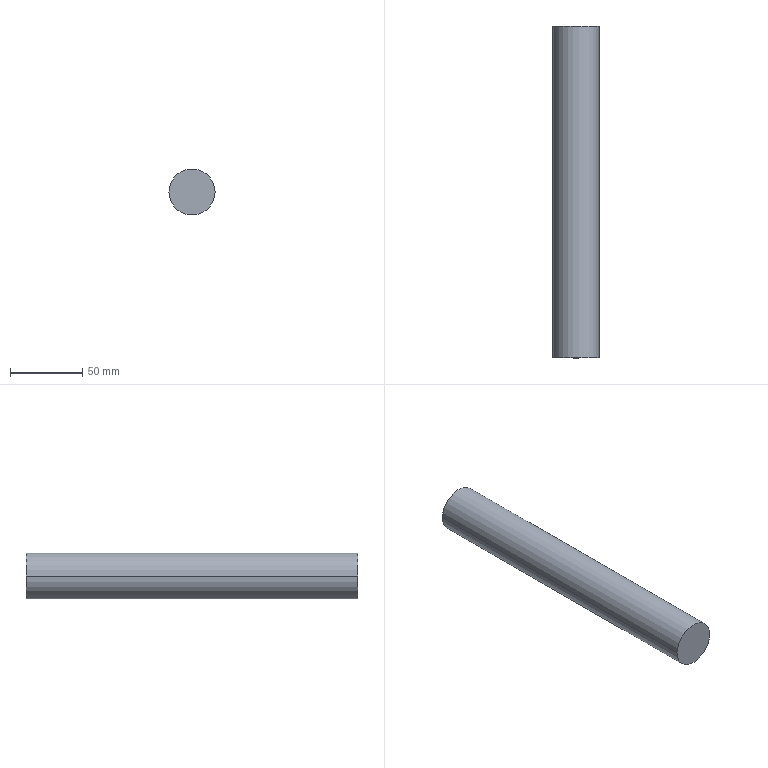Component | SolidWorks | Part1^CentrifugalDehydrator-1 | 1 solid | 4 faces | box 31.75 x 229 x 31.75 mm | volume 181306 mm3 | cylinder 2 | plane 2 | commonest cylinder face diameters 31.75 x2
STEP:
#1=CARTESIAN_POINT('',(-4.218,-13.938,-16.311));
#2=VERTEX_POINT('',#1);
#3=CARTESIAN_POINT('',(-5.468,-13.938,-16.311));
#4=VERTEX_POINT('',#3);
#5=CARTESIAN_POINT('',(-4.843,-13.938,-16.311));
#6=DIRECTION('',(-0.,-1.,-0.));
#7=DIRECTION('',(1.,0.,0.));
#8=AXIS2_PLACEMENT_3D('',#5,#6,#7);
#9=CIRCLE('',#8,0.625);
#10=EDGE_CURVE('',#2,#4,#9,.T.);
#11=ORIENTED_EDGE('',*,*,#10,.T.);
#12=CARTESIAN_POINT('',(-5.468,-22.953,-16.311));
#13=VERTEX_POINT('',#12);
#14=CARTESIAN_POINT('',(-5.468,-13.938,-16.311));
#15=DIRECTION('',(-0.,-1.,-0.));
#16=VECTOR('',#15,39.37);
#17=LINE('',#14,#16);
#18=EDGE_CURVE('',#4,#13,#17,.T.);
#19=ORIENTED_EDGE('',*,*,#18,.T.);
#20=CARTESIAN_POINT('',(-4.218,-22.953,-16.311));
#21=VERTEX_POINT('',#20);
#22=CARTESIAN_POINT('',(-4.843,-22.953,-16.311));
#23=DIRECTION('',(-0.,-1.,-0.));
#24=DIRECTION('',(1.,0.,0.));
#25=AXIS2_PLACEMENT_3D('',#22,#23,#24);
#26=CIRCLE('',#25,0.625);
#27=EDGE_CURVE('',#21,#13,#26,.T.);
#28=ORIENTED_EDGE('',*,*,#27,.F.);
#29=CARTESIAN_POINT('',(-4.218,-13.938,-16.311));
#30=DIRECTION('',(-0.,-1.,-0.));
#31=VECTOR('',#30,39.37);
#32=LINE('',#29,#31);
#33=EDGE_CURVE('',#2,#21,#32,.T.);
#34=ORIENTED_EDGE('',*,*,#33,.F.);
#35=EDGE_LOOP('',(#11,#19,#28,#34));
#36=FACE_OUTER_BOUND('',#35,.T.);
#37=CARTESIAN_POINT('',(-4.843,-13.938,-16.311));
#38=DIRECTION('',(-0.,-1.,-0.));
#39=DIRECTION('',(1.,0.,0.));
#40=AXIS2_PLACEMENT_3D('',#37,#38,#39);
#41=CYLINDRICAL_SURFACE('',#40,0.625);
#42=ADVANCED_FACE('',(#36),#41,.T.);
#43=ORIENTED_EDGE('',*,*,#18,.F.);
#44=CARTESIAN_POINT('',(-4.843,-13.938,-16.311));
#45=DIRECTION('',(-0.,-1.,-0.));
#46=DIRECTION('',(1.,0.,0.));
#47=AXIS2_PLACEMENT_3D('',#44,#45,#46);
#48=CIRCLE('',#47,0.625);
#49=EDGE_CURVE('',#4,#2,#48,.T.);
#50=ORIENTED_EDGE('',*,*,#49,.T.);
#51=ORIENTED_EDGE('',*,*,#33,.T.);
#52=CARTESIAN_POINT('',(-4.843,-22.953,-16.311));
#53=DIRECTION('',(-0.,-1.,-0.));
#54=DIRECTION('',(1.,0.,0.));
#55=AXIS2_PLACEMENT_3D('',#52,#53,#54);
#56=CIRCLE('',#55,0.625);
#57=EDGE_CURVE('',#13,#21,#56,.T.);
#58=ORIENTED_EDGE('',*,*,#57,.F.);
#59=EDGE_LOOP('',(#43,#50,#51,#58));
#60=FACE_OUTER_BOUND('',#59,.T.);
#61=CARTESIAN_POINT('',(-4.843,-13.938,-16.311));
#62=DIRECTION('',(-0.,-1.,-0.));
#63=DIRECTION('',(1.,0.,0.));
#64=AXIS2_PLACEMENT_3D('',#61,#62,#63);
#65=CYLINDRICAL_SURFACE('',#64,0.625);
#66=ADVANCED_FACE('',(#60),#65,.T.);
#67=ORIENTED_EDGE('',*,*,#10,.F.);
#68=ORIENTED_EDGE('',*,*,#49,.F.);
#69=EDGE_LOOP('',(#67,#68));
#70=FACE_OUTER_BOUND('',#69,.T.);
#71=CARTESIAN_POINT('',(-4.843,-13.938,-16.311));
#72=DIRECTION('',(0.,-1.,-0.));
#73=DIRECTION('',(1.,0.,0.));
#74=AXIS2_PLACEMENT_3D('',#71,#72,#73);
#75=PLANE('',#74);
#76=ADVANCED_FACE('',(#70),#75,.F.);
#77=ORIENTED_EDGE('',*,*,#27,.T.);
#78=ORIENTED_EDGE('',*,*,#57,.T.);
#79=EDGE_LOOP('',(#77,#78));
#80=FACE_OUTER_BOUND('',#79,.T.);
#81=CARTESIAN_POINT('',(-4.843,-22.953,-16.311));
#82=DIRECTION('',(0.,-1.,-0.));
#83=DIRECTION('',(1.,0.,0.));
#84=AXIS2_PLACEMENT_3D('',#81,#82,#83);
#85=PLANE('',#84);
#86=ADVANCED_FACE('',(#80),#85,.T.);
#87=CLOSED_SHELL('',(#42,#66,#76,#86));
#88=MANIFOLD_SOLID_BREP('',#87);
#89=CARTESIAN_POINT('',(0.,0.,0.));
#90=DIRECTION('',(0.,0.,1.));
#91=DIRECTION('',(1.,0.,0.));
#92=AXIS2_PLACEMENT_3D('',#89,#90,#91);
#93=(LENGTH_UNIT()NAMED_UNIT(*)SI_UNIT($,.METRE.));
#94=LENGTH_MEASURE_WITH_UNIT(LENGTH_MEASURE(0.0254),#93);
#95=DIMENSIONAL_EXPONENTS(1.,0.,0.,0.,0.,0.,0.);
#96=(CONVERSION_BASED_UNIT('',#94)LENGTH_UNIT()NAMED_UNIT(#95));
#97=UNCERTAINTY_MEASURE_WITH_UNIT(LENGTH_MEASURE(0.00001),#96,'','');
#98=(NAMED_UNIT(*)PLANE_ANGLE_UNIT()SI_UNIT($,.RADIAN.));
#99=(NAMED_UNIT(*)SI_UNIT($,.STERADIAN.)SOLID_ANGLE_UNIT());
#100=(GEOMETRIC_REPRESENTATION_CONTEXT(3)GLOBAL_UNCERTAINTY_ASSIGNED_CONTEXT((#97))GLOBAL_UNIT_ASSIGNED_CONTEXT((#96,#98,#99))REPRESENTATION_CONTEXT('',''));
#101=ADVANCED_BREP_SHAPE_REPRESENTATION('',(#88,#92),#100);
#102=COLOUR_RGB('',0.7922,0.8196,0.9333);
#103=FILL_AREA_STYLE_COLOUR('',#102);
#104=FILL_AREA_STYLE('',(#103));
#105=SURFACE_STYLE_FILL_AREA(#104);
#106=SURFACE_SIDE_STYLE('',(#105));
#107=SURFACE_STYLE_USAGE(.BOTH.,#106);
#108=PRESENTATION_STYLE_ASSIGNMENT((#107));
#109=STYLED_ITEM('',(#108),#88);
#110=(LENGTH_UNIT()NAMED_UNIT(*)SI_UNIT($,.METRE.));
#111=LENGTH_MEASURE_WITH_UNIT(LENGTH_MEASURE(0.0254),#110);
#112=DIMENSIONAL_EXPONENTS(1.,0.,0.,0.,0.,0.,0.);
#113=(CONVERSION_BASED_UNIT('',#111)LENGTH_UNIT()NAMED_UNIT(#112));
#114=UNCERTAINTY_MEASURE_WITH_UNIT(LENGTH_MEASURE(0.00001),#113,'','');
#115=(NAMED_UNIT(*)PLANE_ANGLE_UNIT()SI_UNIT($,.RADIAN.));
#116=(NAMED_UNIT(*)SI_UNIT($,.STERADIAN.)SOLID_ANGLE_UNIT());
#117=(GEOMETRIC_REPRESENTATION_CONTEXT(3)GLOBAL_UNCERTAINTY_ASSIGNED_CONTEXT((#114))GLOBAL_UNIT_ASSIGNED_CONTEXT((#113,#115,#116))REPRESENTATION_CONTEXT('',''));
#118=MECHANICAL_DESIGN_GEOMETRIC_PRESENTATION_REPRESENTATION('',(#109),#117);
#119=PRESENTATION_LAYER_ASSIGNMENT('','',(#109));